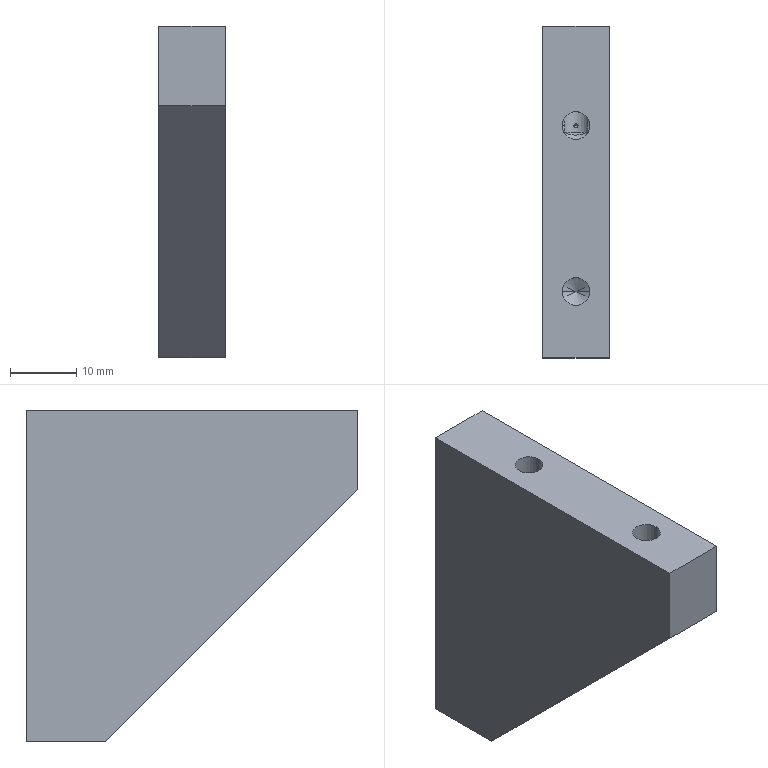Component | SolidWorks | LD101-02--Q1070-Q1-2-2 | 1 solid | 37 faces | box 10 x 50 x 50 mm | volume 16911 mm3 | cone 16 | cylinder 14 | plane 7 | commonest cylinder face diameters 4.2 x14 | material AL6061
STEP:
#1=CARTESIAN_POINT('',(6.957,-10.991,10.561));
#2=VERTEX_POINT('',#1);
#3=CARTESIAN_POINT('',(6.969,-10.983,10.561));
#4=VERTEX_POINT('',#3);
#5=CARTESIAN_POINT('',(7.04,-10.941,10.561));
#6=DIRECTION('',(0.8572,0.515,0.));
#7=VECTOR('',#6,39.37);
#8=LINE('',#5,#7);
#9=EDGE_CURVE('',#2,#4,#8,.T.);
#10=ORIENTED_EDGE('',*,*,#9,.F.);
#11=CARTESIAN_POINT('',(6.945,-10.983,10.561));
#12=VERTEX_POINT('',#11);
#13=CARTESIAN_POINT('',(6.874,-10.941,10.561));
#14=DIRECTION('',(-0.8572,0.515,-0.));
#15=VECTOR('',#14,39.37);
#16=LINE('',#13,#15);
#17=EDGE_CURVE('',#2,#12,#16,.T.);
#18=ORIENTED_EDGE('',*,*,#17,.T.);
#19=CARTESIAN_POINT('',(6.945,-10.983,10.561));
#20=CARTESIAN_POINT('',(6.945,-10.983,10.564));
#21=CARTESIAN_POINT('',(6.947,-10.983,10.567));
#22=CARTESIAN_POINT('',(6.951,-10.984,10.571));
#23=CARTESIAN_POINT('',(6.954,-10.984,10.572));
#24=CARTESIAN_POINT('',(6.96,-10.984,10.572));
#25=CARTESIAN_POINT('',(6.963,-10.984,10.571));
#26=CARTESIAN_POINT('',(6.968,-10.983,10.567));
#27=CARTESIAN_POINT('',(6.969,-10.983,10.564));
#28=CARTESIAN_POINT('',(6.969,-10.983,10.561));
#29=B_SPLINE_CURVE_WITH_KNOTS('',3,(#19,#20,#21,#22,#23,#24,#25,#26,#27,#28),.UNSPECIFIED.,.F.,.F.,(4,2,2,2,4),(0.000232,0.0004572,0.0006825,0.0009077,0.001133),.UNSPECIFIED.);
#30=EDGE_CURVE('',#12,#4,#29,.T.);
#31=ORIENTED_EDGE('',*,*,#30,.T.);
#32=EDGE_LOOP('',(#10,#18,#31));
#33=FACE_OUTER_BOUND('',#32,.T.);
#34=CARTESIAN_POINT('',(6.957,-10.941,10.561));
#35=DIRECTION('',(-0.,1.,-0.));
#36=DIRECTION('',(1.,0.,0.));
#37=AXIS2_PLACEMENT_3D('',#34,#35,#36);
#38=CONICAL_SURFACE('',#37,0.08268,1.03);
#39=ADVANCED_FACE('',(#33),#38,.F.);
#40=CARTESIAN_POINT('',(7.04,-10.941,10.561));
#41=VERTEX_POINT('',#40);
#42=CARTESIAN_POINT('',(7.03,-10.941,10.522));
#43=VERTEX_POINT('',#42);
#44=CARTESIAN_POINT('',(6.957,-10.941,10.561));
#45=DIRECTION('',(-0.,1.,-0.));
#46=DIRECTION('',(1.,0.,0.));
#47=AXIS2_PLACEMENT_3D('',#44,#45,#46);
#48=CIRCLE('',#47,0.08268);
#49=EDGE_CURVE('',#41,#43,#48,.T.);
#50=ORIENTED_EDGE('',*,*,#49,.F.);
#51=CARTESIAN_POINT('',(7.04,-10.901,10.561));
#52=VERTEX_POINT('',#51);
#53=CARTESIAN_POINT('',(7.04,-10.311,10.561));
#54=DIRECTION('',(-0.,1.,-0.));
#55=VECTOR('',#54,39.37);
#56=LINE('',#53,#55);
#57=EDGE_CURVE('',#41,#52,#56,.T.);
#58=ORIENTED_EDGE('',*,*,#57,.T.);
#59=CARTESIAN_POINT('',(7.04,-10.901,10.561));
#60=CARTESIAN_POINT('',(7.04,-10.915,10.547));
#61=CARTESIAN_POINT('',(7.036,-10.929,10.534));
#62=CARTESIAN_POINT('',(7.03,-10.941,10.522));
#63=(BOUNDED_CURVE()B_SPLINE_CURVE(3,(#59,#60,#61,#62),.UNSPECIFIED.,.F.,.F.)B_SPLINE_CURVE_WITH_KNOTS((4,4),(1.571,2.067),.UNSPECIFIED.)CURVE()GEOMETRIC_REPRESENTATION_ITEM()RATIONAL_B_SPLINE_CURVE((1.,0.9796,0.9796,1.))REPRESENTATION_ITEM(''));
#64=EDGE_CURVE('',#52,#43,#63,.T.);
#65=ORIENTED_EDGE('',*,*,#64,.T.);
#66=EDGE_LOOP('',(#50,#58,#65));
#67=FACE_OUTER_BOUND('',#66,.T.);
#68=CARTESIAN_POINT('',(6.957,-10.311,10.561));
#69=DIRECTION('',(-0.,1.,-0.));
#70=DIRECTION('',(1.,0.,0.));
#71=AXIS2_PLACEMENT_3D('',#68,#69,#70);
#72=CYLINDRICAL_SURFACE('',#71,0.08268);
#73=ADVANCED_FACE('',(#67),#72,.F.);
#74=CARTESIAN_POINT('',(7.024,-10.951,10.561));
#75=VERTEX_POINT('',#74);
#76=CARTESIAN_POINT('',(7.03,-10.941,10.522));
#77=CARTESIAN_POINT('',(7.028,-10.943,10.528));
#78=CARTESIAN_POINT('',(7.027,-10.946,10.534));
#79=CARTESIAN_POINT('',(7.025,-10.948,10.544));
#80=CARTESIAN_POINT('',(7.025,-10.949,10.547));
#81=CARTESIAN_POINT('',(7.024,-10.95,10.554));
#82=CARTESIAN_POINT('',(7.024,-10.951,10.558));
#83=CARTESIAN_POINT('',(7.024,-10.951,10.561));
#84=B_SPLINE_CURVE_WITH_KNOTS('',3,(#76,#77,#78,#79,#80,#81,#82,#83),.UNSPECIFIED.,.F.,.F.,(4,2,2,4),(0.0002892,0.00081,0.00107,0.001331),.UNSPECIFIED.);
#85=EDGE_CURVE('',#43,#75,#84,.T.);
#86=ORIENTED_EDGE('',*,*,#85,.T.);
#87=CARTESIAN_POINT('',(7.04,-10.941,10.561));
#88=DIRECTION('',(0.8572,0.515,0.));
#89=VECTOR('',#88,39.37);
#90=LINE('',#87,#89);
#91=EDGE_CURVE('',#75,#41,#90,.T.);
#92=ORIENTED_EDGE('',*,*,#91,.T.);
#93=ORIENTED_EDGE('',*,*,#49,.T.);
#94=EDGE_LOOP('',(#86,#92,#93));
#95=FACE_OUTER_BOUND('',#94,.T.);
#96=CARTESIAN_POINT('',(6.957,-10.941,10.561));
#97=DIRECTION('',(-0.,1.,-0.));
#98=DIRECTION('',(1.,0.,0.));
#99=AXIS2_PLACEMENT_3D('',#96,#97,#98);
#100=CONICAL_SURFACE('',#99,0.08268,1.03);
#101=ADVANCED_FACE('',(#95),#100,.F.);
#102=CARTESIAN_POINT('',(6.874,-10.901,10.561));
#103=VERTEX_POINT('',#102);
#104=CARTESIAN_POINT('',(7.04,-10.901,10.561));
#105=CARTESIAN_POINT('',(7.04,-10.736,10.727));
#106=CARTESIAN_POINT('',(6.874,-10.736,10.727));
#107=CARTESIAN_POINT('',(6.874,-10.901,10.561));
#108=(BOUNDED_CURVE()B_SPLINE_CURVE(3,(#104,#105,#106,#107),.UNSPECIFIED.,.F.,.F.)B_SPLINE_CURVE_WITH_KNOTS((4,4),(4.712,7.854),.UNSPECIFIED.)CURVE()GEOMETRIC_REPRESENTATION_ITEM()RATIONAL_B_SPLINE_CURVE((1.,0.3333,0.3333,1.))REPRESENTATION_ITEM(''));
#109=EDGE_CURVE('',#52,#103,#108,.T.);
#110=ORIENTED_EDGE('',*,*,#109,.F.);
#111=CARTESIAN_POINT('',(7.04,-10.901,11.152));
#112=VERTEX_POINT('',#111);
#113=CARTESIAN_POINT('',(7.04,-10.901,11.152));
#114=DIRECTION('',(-0.,0.,1.));
#115=VECTOR('',#114,39.37);
#116=LINE('',#113,#115);
#117=EDGE_CURVE('',#52,#112,#116,.T.);
#118=ORIENTED_EDGE('',*,*,#117,.T.);
#119=CARTESIAN_POINT('',(6.874,-10.901,11.152));
#120=VERTEX_POINT('',#119);
#121=CARTESIAN_POINT('',(6.957,-10.901,11.152));
#122=DIRECTION('',(-0.,0.,1.));
#123=DIRECTION('',(-1.,0.,0.));
#124=AXIS2_PLACEMENT_3D('',#121,#122,#123);
#125=CIRCLE('',#124,0.08268);
#126=EDGE_CURVE('',#112,#120,#125,.T.);
#127=ORIENTED_EDGE('',*,*,#126,.T.);
#128=CARTESIAN_POINT('',(6.874,-10.901,11.152));
#129=DIRECTION('',(-0.,0.,1.));
#130=VECTOR('',#129,39.37);
#131=LINE('',#128,#130);
#132=EDGE_CURVE('',#103,#120,#131,.T.);
#133=ORIENTED_EDGE('',*,*,#132,.F.);
#134=EDGE_LOOP('',(#110,#118,#127,#133));
#135=FACE_OUTER_BOUND('',#134,.T.);
#136=CARTESIAN_POINT('',(6.957,-10.901,11.152));
#137=DIRECTION('',(-0.,0.,1.));
#138=DIRECTION('',(-1.,0.,0.));
#139=AXIS2_PLACEMENT_3D('',#136,#137,#138);
#140=CYLINDRICAL_SURFACE('',#139,0.08268);
#141=ADVANCED_FACE('',(#135),#140,.F.);
#142=CARTESIAN_POINT('',(6.874,-10.901,10.522));
#143=VERTEX_POINT('',#142);
#144=CARTESIAN_POINT('',(6.884,-10.941,10.522));
#145=VERTEX_POINT('',#144);
#146=CARTESIAN_POINT('',(6.957,-10.901,10.522));
#147=DIRECTION('',(-0.,0.,1.));
#148=DIRECTION('',(-1.,0.,0.));
#149=AXIS2_PLACEMENT_3D('',#146,#147,#148);
#150=CIRCLE('',#149,0.08268);
#151=EDGE_CURVE('',#143,#145,#150,.T.);
#152=ORIENTED_EDGE('',*,*,#151,.F.);
#153=CARTESIAN_POINT('',(6.874,-10.901,11.152));
#154=DIRECTION('',(-0.,0.,1.));
#155=VECTOR('',#154,39.37);
#156=LINE('',#153,#155);
#157=EDGE_CURVE('',#143,#103,#156,.T.);
#158=ORIENTED_EDGE('',*,*,#157,.T.);
#159=CARTESIAN_POINT('',(6.884,-10.941,10.522));
#160=CARTESIAN_POINT('',(6.878,-10.929,10.534));
#161=CARTESIAN_POINT('',(6.874,-10.915,10.547));
#162=CARTESIAN_POINT('',(6.874,-10.901,10.561));
#163=(BOUNDED_CURVE()B_SPLINE_CURVE(3,(#159,#160,#161,#162),.UNSPECIFIED.,.F.,.F.)B_SPLINE_CURVE_WITH_KNOTS((4,4),(4.216,4.712),.UNSPECIFIED.)CURVE()GEOMETRIC_REPRESENTATION_ITEM()RATIONAL_B_SPLINE_CURVE((1.,0.9796,0.9796,1.))REPRESENTATION_ITEM(''));
#164=EDGE_CURVE('',#145,#103,#163,.T.);
#165=ORIENTED_EDGE('',*,*,#164,.F.);
#166=EDGE_LOOP('',(#152,#158,#165));
#167=FACE_OUTER_BOUND('',#166,.T.);
#168=CARTESIAN_POINT('',(6.957,-10.901,11.152));
#169=DIRECTION('',(-0.,0.,1.));
#170=DIRECTION('',(-1.,0.,0.));
#171=AXIS2_PLACEMENT_3D('',#168,#169,#170);
#172=CYLINDRICAL_SURFACE('',#171,0.08268);
#173=ADVANCED_FACE('',(#167),#172,.F.);
#174=CARTESIAN_POINT('',(6.891,-10.901,10.512));
#175=VERTEX_POINT('',#174);
#176=CARTESIAN_POINT('',(6.891,-10.901,10.512));
#177=CARTESIAN_POINT('',(6.891,-10.908,10.512));
#178=CARTESIAN_POINT('',(6.89,-10.915,10.513));
#179=CARTESIAN_POINT('',(6.887,-10.928,10.517));
#180=CARTESIAN_POINT('',(6.886,-10.935,10.519));
#181=CARTESIAN_POINT('',(6.884,-10.941,10.522));
#182=B_SPLINE_CURVE_WITH_KNOTS('',3,(#176,#177,#178,#179,#180,#181),.UNSPECIFIED.,.F.,.F.,(4,2,4),(0.001331,0.001845,0.00236),.UNSPECIFIED.);
#183=EDGE_CURVE('',#175,#145,#182,.T.);
#184=ORIENTED_EDGE('',*,*,#183,.F.);
#185=CARTESIAN_POINT('',(6.874,-10.901,10.522));
#186=DIRECTION('',(-0.8572,0.,0.515));
#187=VECTOR('',#186,39.37);
#188=LINE('',#185,#187);
#189=EDGE_CURVE('',#175,#143,#188,.T.);
#190=ORIENTED_EDGE('',*,*,#189,.T.);
#191=ORIENTED_EDGE('',*,*,#151,.T.);
#192=EDGE_LOOP('',(#184,#190,#191));
#193=FACE_OUTER_BOUND('',#192,.T.);
#194=CARTESIAN_POINT('',(6.957,-10.901,10.522));
#195=DIRECTION('',(-0.,0.,1.));
#196=DIRECTION('',(-1.,0.,0.));
#197=AXIS2_PLACEMENT_3D('',#194,#195,#196);
#198=CONICAL_SURFACE('',#197,0.08268,1.03);
#199=ADVANCED_FACE('',(#193),#198,.F.);
#200=CARTESIAN_POINT('',(6.957,-10.901,10.472));
#201=VERTEX_POINT('',#200);
#202=CARTESIAN_POINT('',(6.945,-10.901,10.479));
#203=VERTEX_POINT('',#202);
#204=CARTESIAN_POINT('',(6.874,-10.901,10.522));
#205=DIRECTION('',(-0.8572,0.,0.515));
#206=VECTOR('',#205,39.37);
#207=LINE('',#204,#206);
#208=EDGE_CURVE('',#201,#203,#207,.T.);
#209=ORIENTED_EDGE('',*,*,#208,.F.);
#210=CARTESIAN_POINT('',(6.969,-10.901,10.479));
#211=VERTEX_POINT('',#210);
#212=CARTESIAN_POINT('',(7.04,-10.901,10.522));
#213=DIRECTION('',(0.8572,0.,0.515));
#214=VECTOR('',#213,39.37);
#215=LINE('',#212,#214);
#216=EDGE_CURVE('',#201,#211,#215,.T.);
#217=ORIENTED_EDGE('',*,*,#216,.T.);
#218=CARTESIAN_POINT('',(6.945,-10.901,10.479));
#219=CARTESIAN_POINT('',(6.945,-10.898,10.479));
#220=CARTESIAN_POINT('',(6.947,-10.896,10.479));
#221=CARTESIAN_POINT('',(6.951,-10.892,10.479));
#222=CARTESIAN_POINT('',(6.954,-10.891,10.479));
#223=CARTESIAN_POINT('',(6.96,-10.891,10.479));
#224=CARTESIAN_POINT('',(6.963,-10.892,10.479));
#225=CARTESIAN_POINT('',(6.968,-10.896,10.479));
#226=CARTESIAN_POINT('',(6.969,-10.898,10.479));
#227=CARTESIAN_POINT('',(6.969,-10.901,10.479));
#228=B_SPLINE_CURVE_WITH_KNOTS('',3,(#218,#219,#220,#221,#222,#223,#224,#225,#226,#227),.UNSPECIFIED.,.F.,.F.,(4,2,2,2,4),(0.000232,0.0004572,0.0006825,0.0009077,0.001133),.UNSPECIFIED.);
#229=EDGE_CURVE('',#203,#211,#228,.T.);
#230=ORIENTED_EDGE('',*,*,#229,.F.);
#231=EDGE_LOOP('',(#209,#217,#230));
#232=FACE_OUTER_BOUND('',#231,.T.);
#233=CARTESIAN_POINT('',(6.957,-10.901,10.522));
#234=DIRECTION('',(-0.,0.,1.));
#235=DIRECTION('',(-1.,0.,0.));
#236=AXIS2_PLACEMENT_3D('',#233,#234,#235);
#237=CONICAL_SURFACE('',#236,0.08268,1.03);
#238=ADVANCED_FACE('',(#232),#237,.F.);
#239=CARTESIAN_POINT('',(7.04,-11.886,10.522));
#240=VERTEX_POINT('',#239);
#241=CARTESIAN_POINT('',(6.874,-11.886,10.522));
#242=VERTEX_POINT('',#241);
#243=CARTESIAN_POINT('',(6.957,-11.886,10.522));
#244=DIRECTION('',(-0.,0.,1.));
#245=DIRECTION('',(-1.,0.,0.));
#246=AXIS2_PLACEMENT_3D('',#243,#244,#245);
#247=CIRCLE('',#246,0.08268);
#248=EDGE_CURVE('',#240,#242,#247,.T.);
#249=ORIENTED_EDGE('',*,*,#248,.F.);
#250=CARTESIAN_POINT('',(7.04,-11.886,11.152));
#251=VERTEX_POINT('',#250);
#252=CARTESIAN_POINT('',(7.04,-11.886,11.152));
#253=DIRECTION('',(-0.,0.,1.));
#254=VECTOR('',#253,39.37);
#255=LINE('',#252,#254);
#256=EDGE_CURVE('',#240,#251,#255,.T.);
#257=ORIENTED_EDGE('',*,*,#256,.T.);
#258=CARTESIAN_POINT('',(6.874,-11.886,11.152));
#259=VERTEX_POINT('',#258);
#260=CARTESIAN_POINT('',(6.957,-11.886,11.152));
#261=DIRECTION('',(-0.,0.,1.));
#262=DIRECTION('',(-1.,0.,0.));
#263=AXIS2_PLACEMENT_3D('',#260,#261,#262);
#264=CIRCLE('',#263,0.08268);
#265=EDGE_CURVE('',#251,#259,#264,.T.);
#266=ORIENTED_EDGE('',*,*,#265,.T.);
#267=CARTESIAN_POINT('',(6.874,-11.886,11.152));
#268=DIRECTION('',(-0.,0.,1.));
#269=VECTOR('',#268,39.37);
#270=LINE('',#267,#269);
#271=EDGE_CURVE('',#242,#259,#270,.T.);
#272=ORIENTED_EDGE('',*,*,#271,.F.);
#273=EDGE_LOOP('',(#249,#257,#266,#272));
#274=FACE_OUTER_BOUND('',#273,.T.);
#275=CARTESIAN_POINT('',(6.957,-11.886,11.152));
#276=DIRECTION('',(-0.,0.,1.));
#277=DIRECTION('',(-1.,0.,0.));
#278=AXIS2_PLACEMENT_3D('',#275,#276,#277);
#279=CYLINDRICAL_SURFACE('',#278,0.08268);
#280=ADVANCED_FACE('',(#274),#279,.F.);
#281=CARTESIAN_POINT('',(6.957,-11.886,10.472));
#282=VERTEX_POINT('',#281);
#283=CARTESIAN_POINT('',(6.874,-11.886,10.522));
#284=DIRECTION('',(-0.8572,0.,0.515));
#285=VECTOR('',#284,39.37);
#286=LINE('',#283,#285);
#287=EDGE_CURVE('',#282,#242,#286,.T.);
#288=ORIENTED_EDGE('',*,*,#287,.F.);
#289=CARTESIAN_POINT('',(7.04,-11.886,10.522));
#290=DIRECTION('',(0.8572,0.,0.515));
#291=VECTOR('',#290,39.37);
#292=LINE('',#289,#291);
#293=EDGE_CURVE('',#282,#240,#292,.T.);
#294=ORIENTED_EDGE('',*,*,#293,.T.);
#295=ORIENTED_EDGE('',*,*,#248,.T.);
#296=EDGE_LOOP('',(#288,#294,#295));
#297=FACE_OUTER_BOUND('',#296,.T.);
#298=CARTESIAN_POINT('',(6.957,-11.886,10.522));
#299=DIRECTION('',(-0.,0.,1.));
#300=DIRECTION('',(-1.,0.,0.));
#301=AXIS2_PLACEMENT_3D('',#298,#299,#300);
#302=CONICAL_SURFACE('',#301,0.08268,1.03);
#303=ADVANCED_FACE('',(#297),#302,.F.);
#304=CARTESIAN_POINT('',(6.874,-10.941,9.577));
#305=VERTEX_POINT('',#304);
#306=CARTESIAN_POINT('',(7.04,-10.941,9.577));
#307=VERTEX_POINT('',#306);
#308=CARTESIAN_POINT('',(6.957,-10.941,9.577));
#309=DIRECTION('',(-0.,1.,-0.));
#310=DIRECTION('',(1.,0.,0.));
#311=AXIS2_PLACEMENT_3D('',#308,#309,#310);
#312=CIRCLE('',#311,0.08268);
#313=EDGE_CURVE('',#305,#307,#312,.T.);
#314=ORIENTED_EDGE('',*,*,#313,.F.);
#315=CARTESIAN_POINT('',(6.874,-10.311,9.577));
#316=VERTEX_POINT('',#315);
#317=CARTESIAN_POINT('',(6.874,-10.311,9.577));
#318=DIRECTION('',(-0.,1.,-0.));
#319=VECTOR('',#318,39.37);
#320=LINE('',#317,#319);
#321=EDGE_CURVE('',#305,#316,#320,.T.);
#322=ORIENTED_EDGE('',*,*,#321,.T.);
#323=CARTESIAN_POINT('',(7.04,-10.311,9.577));
#324=VERTEX_POINT('',#323);
#325=CARTESIAN_POINT('',(6.957,-10.311,9.577));
#326=DIRECTION('',(-0.,1.,-0.));
#327=DIRECTION('',(1.,0.,0.));
#328=AXIS2_PLACEMENT_3D('',#325,#326,#327);
#329=CIRCLE('',#328,0.08268);
#330=EDGE_CURVE('',#316,#324,#329,.T.);
#331=ORIENTED_EDGE('',*,*,#330,.T.);
#332=CARTESIAN_POINT('',(7.04,-10.311,9.577));
#333=DIRECTION('',(-0.,1.,-0.));
#334=VECTOR('',#333,39.37);
#335=LINE('',#332,#334);
#336=EDGE_CURVE('',#307,#324,#335,.T.);
#337=ORIENTED_EDGE('',*,*,#336,.F.);
#338=EDGE_LOOP('',(#314,#322,#331,#337));
#339=FACE_OUTER_BOUND('',#338,.T.);
#340=CARTESIAN_POINT('',(6.957,-10.311,9.577));
#341=DIRECTION('',(-0.,1.,-0.));
#342=DIRECTION('',(1.,0.,0.));
#343=AXIS2_PLACEMENT_3D('',#340,#341,#342);
#344=CYLINDRICAL_SURFACE('',#343,0.08268);
#345=ADVANCED_FACE('',(#339),#344,.F.);
#346=CARTESIAN_POINT('',(6.957,-10.991,9.577));
#347=VERTEX_POINT('',#346);
#348=CARTESIAN_POINT('',(7.04,-10.941,9.577));
#349=DIRECTION('',(0.8572,0.515,0.));
#350=VECTOR('',#349,39.37);
#351=LINE('',#348,#350);
#352=EDGE_CURVE('',#347,#307,#351,.T.);
#353=ORIENTED_EDGE('',*,*,#352,.F.);
#354=CARTESIAN_POINT('',(6.874,-10.941,9.577));
#355=DIRECTION('',(-0.8572,0.515,-0.));
#356=VECTOR('',#355,39.37);
#357=LINE('',#354,#356);
#358=EDGE_CURVE('',#347,#305,#357,.T.);
#359=ORIENTED_EDGE('',*,*,#358,.T.);
#360=ORIENTED_EDGE('',*,*,#313,.T.);
#361=EDGE_LOOP('',(#353,#359,#360));
#362=FACE_OUTER_BOUND('',#361,.T.);
#363=CARTESIAN_POINT('',(6.957,-10.941,9.577));
#364=DIRECTION('',(-0.,1.,-0.));
#365=DIRECTION('',(1.,0.,0.));
#366=AXIS2_PLACEMENT_3D('',#363,#364,#365);
#367=CONICAL_SURFACE('',#366,0.08268,1.03);
#368=ADVANCED_FACE('',(#362),#367,.F.);
#369=ORIENTED_EDGE('',*,*,#109,.T.);
#370=CARTESIAN_POINT('',(6.874,-10.311,10.561));
#371=VERTEX_POINT('',#370);
#372=CARTESIAN_POINT('',(6.874,-10.311,10.561));
#373=DIRECTION('',(-0.,1.,-0.));
#374=VECTOR('',#373,39.37);
#375=LINE('',#372,#374);
#376=EDGE_CURVE('',#103,#371,#375,.T.);
#377=ORIENTED_EDGE('',*,*,#376,.T.);
#378=CARTESIAN_POINT('',(7.04,-10.311,10.561));
#379=VERTEX_POINT('',#378);
#380=CARTESIAN_POINT('',(6.957,-10.311,10.561));
#381=DIRECTION('',(-0.,1.,-0.));
#382=DIRECTION('',(1.,0.,0.));
#383=AXIS2_PLACEMENT_3D('',#380,#381,#382);
#384=CIRCLE('',#383,0.08268);
#385=EDGE_CURVE('',#371,#379,#384,.T.);
#386=ORIENTED_EDGE('',*,*,#385,.T.);
#387=CARTESIAN_POINT('',(7.04,-10.311,10.561));
#388=DIRECTION('',(-0.,1.,-0.));
#389=VECTOR('',#388,39.37);
#390=LINE('',#387,#389);
#391=EDGE_CURVE('',#52,#379,#390,.T.);
#392=ORIENTED_EDGE('',*,*,#391,.F.);
#393=EDGE_LOOP('',(#369,#377,#386,#392));
#394=FACE_OUTER_BOUND('',#393,.T.);
#395=CARTESIAN_POINT('',(6.957,-10.311,10.561));
#396=DIRECTION('',(-0.,1.,-0.));
#397=DIRECTION('',(1.,0.,0.));
#398=AXIS2_PLACEMENT_3D('',#395,#396,#397);
#399=CYLINDRICAL_SURFACE('',#398,0.08268);
#400=ADVANCED_FACE('',(#394),#399,.F.);
#401=CARTESIAN_POINT('',(6.957,-10.941,10.561));
#402=DIRECTION('',(-0.,1.,-0.));
#403=DIRECTION('',(1.,0.,0.));
#404=AXIS2_PLACEMENT_3D('',#401,#402,#403);
#405=CIRCLE('',#404,0.08268);
#406=EDGE_CURVE('',#43,#145,#405,.T.);
#407=ORIENTED_EDGE('',*,*,#406,.T.);
#408=CARTESIAN_POINT('',(6.884,-10.941,10.522));
#409=CARTESIAN_POINT('',(6.896,-10.945,10.517));
#410=CARTESIAN_POINT('',(6.907,-10.949,10.513));
#411=CARTESIAN_POINT('',(6.925,-10.954,10.509));
#412=CARTESIAN_POINT('',(6.931,-10.955,10.508));
#413=CARTESIAN_POINT('',(6.944,-10.957,10.506));
#414=CARTESIAN_POINT('',(6.951,-10.957,10.506));
#415=CARTESIAN_POINT('',(6.963,-10.957,10.506));
#416=CARTESIAN_POINT('',(6.97,-10.957,10.506));
#417=CARTESIAN_POINT('',(6.983,-10.955,10.508));
#418=CARTESIAN_POINT('',(6.989,-10.954,10.509));
#419=CARTESIAN_POINT('',(7.007,-10.949,10.513));
#420=CARTESIAN_POINT('',(7.019,-10.945,10.517));
#421=CARTESIAN_POINT('',(7.03,-10.941,10.522));
#422=B_SPLINE_CURVE_WITH_KNOTS('',3,(#408,#409,#410,#411,#412,#413,#414,#415,#416,#417,#418,#419,#420,#421),.UNSPECIFIED.,.F.,.F.,(4,2,2,2,2,2,4),(0.00000056,0.00097,0.001455,0.001939,0.002424,0.002909,0.003878),.UNSPECIFIED.);
#423=EDGE_CURVE('',#145,#43,#422,.T.);
#424=ORIENTED_EDGE('',*,*,#423,.T.);
#425=EDGE_LOOP('',(#407,#424));
#426=FACE_OUTER_BOUND('',#425,.T.);
#427=CARTESIAN_POINT('',(6.957,-10.941,10.561));
#428=DIRECTION('',(-0.,1.,-0.));
#429=DIRECTION('',(1.,0.,0.));
#430=AXIS2_PLACEMENT_3D('',#427,#428,#429);
#431=CONICAL_SURFACE('',#430,0.08268,1.03);
#432=ADVANCED_FACE('',(#426),#431,.F.);
#433=ORIENTED_EDGE('',*,*,#376,.F.);
#434=CARTESIAN_POINT('',(6.884,-10.862,10.522));
#435=VERTEX_POINT('',#434);
#436=CARTESIAN_POINT('',(6.874,-10.901,10.561));
#437=CARTESIAN_POINT('',(6.874,-10.888,10.547));
#438=CARTESIAN_POINT('',(6.878,-10.874,10.534));
#439=CARTESIAN_POINT('',(6.884,-10.862,10.522));
#440=(BOUNDED_CURVE()B_SPLINE_CURVE(3,(#436,#437,#438,#439),.UNSPECIFIED.,.F.,.T.)B_SPLINE_CURVE_WITH_KNOTS((4,4),(4.712,5.209),.UNSPECIFIED.)CURVE()GEOMETRIC_REPRESENTATION_ITEM()RATIONAL_B_SPLINE_CURVE((1.,0.9796,0.9796,1.))REPRESENTATION_ITEM(''));
#441=EDGE_CURVE('',#103,#435,#440,.T.);
#442=ORIENTED_EDGE('',*,*,#441,.T.);
#443=CARTESIAN_POINT('',(6.884,-10.862,10.522));
#444=CARTESIAN_POINT('',(6.886,-10.868,10.519));
#445=CARTESIAN_POINT('',(6.887,-10.875,10.517));
#446=CARTESIAN_POINT('',(6.889,-10.884,10.514));
#447=CARTESIAN_POINT('',(6.89,-10.888,10.514));
#448=CARTESIAN_POINT('',(6.89,-10.894,10.513));
#449=CARTESIAN_POINT('',(6.891,-10.898,10.512));
#450=CARTESIAN_POINT('',(6.891,-10.901,10.512));
#451=B_SPLINE_CURVE_WITH_KNOTS('',3,(#443,#444,#445,#446,#447,#448,#449,#450),.UNSPECIFIED.,.F.,.F.,(4,2,2,4),(0.0002892,0.00081,0.00107,0.001331),.UNSPECIFIED.);
#452=EDGE_CURVE('',#435,#175,#451,.T.);
#453=ORIENTED_EDGE('',*,*,#452,.T.);
#454=ORIENTED_EDGE('',*,*,#183,.T.);
#455=ORIENTED_EDGE('',*,*,#406,.F.);
#456=CARTESIAN_POINT('',(7.03,-10.862,10.522));
#457=VERTEX_POINT('',#456);
#458=CARTESIAN_POINT('',(7.03,-10.941,10.522));
#459=CARTESIAN_POINT('',(7.028,-10.935,10.519));
#460=CARTESIAN_POINT('',(7.027,-10.928,10.517));
#461=CARTESIAN_POINT('',(7.025,-10.919,10.514));
#462=CARTESIAN_POINT('',(7.025,-10.915,10.514));
#463=CARTESIAN_POINT('',(7.024,-10.909,10.513));
#464=CARTESIAN_POINT('',(7.024,-10.905,10.512));
#465=CARTESIAN_POINT('',(7.024,-10.895,10.512));
#466=CARTESIAN_POINT('',(7.025,-10.888,10.513));
#467=CARTESIAN_POINT('',(7.027,-10.875,10.517));
#468=CARTESIAN_POINT('',(7.028,-10.868,10.519));
#469=CARTESIAN_POINT('',(7.03,-10.862,10.522));
#470=B_SPLINE_CURVE_WITH_KNOTS('',3,(#458,#459,#460,#461,#462,#463,#464,#465,#466,#467,#468,#469),.UNSPECIFIED.,.F.,.F.,(4,2,2,2,2,4),(0.0002892,0.0008068,0.001066,0.001324,0.001842,0.00236),.UNSPECIFIED.);
#471=EDGE_CURVE('',#43,#457,#470,.T.);
#472=ORIENTED_EDGE('',*,*,#471,.T.);
#473=CARTESIAN_POINT('',(7.03,-10.862,10.522));
#474=CARTESIAN_POINT('',(7.036,-10.874,10.534));
#475=CARTESIAN_POINT('',(7.04,-10.888,10.547));
#476=CARTESIAN_POINT('',(7.04,-10.901,10.561));
#477=(BOUNDED_CURVE()B_SPLINE_CURVE(3,(#473,#474,#475,#476),.UNSPECIFIED.,.F.,.F.)B_SPLINE_CURVE_WITH_KNOTS((4,4),(1.074,1.571),.UNSPECIFIED.)CURVE()GEOMETRIC_REPRESENTATION_ITEM()RATIONAL_B_SPLINE_CURVE((1.,0.9796,0.9796,1.))REPRESENTATION_ITEM(''));
#478=EDGE_CURVE('',#457,#52,#477,.T.);
#479=ORIENTED_EDGE('',*,*,#478,.T.);
#480=ORIENTED_EDGE('',*,*,#391,.T.);
#481=CARTESIAN_POINT('',(6.957,-10.311,10.561));
#482=DIRECTION('',(-0.,1.,-0.));
#483=DIRECTION('',(1.,0.,0.));
#484=AXIS2_PLACEMENT_3D('',#481,#482,#483);
#485=CIRCLE('',#484,0.08268);
#486=EDGE_CURVE('',#379,#371,#485,.T.);
#487=ORIENTED_EDGE('',*,*,#486,.T.);
#488=EDGE_LOOP('',(#433,#442,#453,#454,#455,#472,#479,#480,#487));
#489=FACE_OUTER_BOUND('',#488,.T.);
#490=ORIENTED_EDGE('',*,*,#229,.T.);
#491=CARTESIAN_POINT('',(6.969,-10.901,10.479));
#492=CARTESIAN_POINT('',(6.969,-10.904,10.479));
#493=CARTESIAN_POINT('',(6.968,-10.907,10.479));
#494=CARTESIAN_POINT('',(6.963,-10.911,10.479));
#495=CARTESIAN_POINT('',(6.96,-10.912,10.479));
#496=CARTESIAN_POINT('',(6.954,-10.912,10.479));
#497=CARTESIAN_POINT('',(6.951,-10.911,10.479));
#498=CARTESIAN_POINT('',(6.947,-10.907,10.479));
#499=CARTESIAN_POINT('',(6.945,-10.904,10.479));
#500=CARTESIAN_POINT('',(6.945,-10.901,10.479));
#501=B_SPLINE_CURVE_WITH_KNOTS('',3,(#491,#492,#493,#494,#495,#496,#497,#498,#499,#500),.UNSPECIFIED.,.F.,.F.,(4,2,2,2,4),(0.001133,0.001358,0.001583,0.001807,0.002032),.UNSPECIFIED.);
#502=EDGE_CURVE('',#211,#203,#501,.T.);
#503=ORIENTED_EDGE('',*,*,#502,.T.);
#504=EDGE_LOOP('',(#490,#503));
#505=FACE_BOUND('',#504,.T.);
#506=CARTESIAN_POINT('',(6.957,-10.311,10.561));
#507=DIRECTION('',(-0.,1.,-0.));
#508=DIRECTION('',(1.,0.,0.));
#509=AXIS2_PLACEMENT_3D('',#506,#507,#508);
#510=CYLINDRICAL_SURFACE('',#509,0.08268);
#511=ADVANCED_FACE('',(#489,#505),#510,.F.);
#512=ORIENTED_EDGE('',*,*,#486,.F.);
#513=ORIENTED_EDGE('',*,*,#385,.F.);
#514=EDGE_LOOP('',(#512,#513));
#515=FACE_BOUND('',#514,.T.);
#516=CARTESIAN_POINT('',(6.957,-10.311,9.577));
#517=DIRECTION('',(-0.,1.,-0.));
#518=DIRECTION('',(1.,0.,0.));
#519=AXIS2_PLACEMENT_3D('',#516,#517,#518);
#520=CIRCLE('',#519,0.08268);
#521=EDGE_CURVE('',#324,#316,#520,.T.);
#522=ORIENTED_EDGE('',*,*,#521,.F.);
#523=ORIENTED_EDGE('',*,*,#330,.F.);
#524=EDGE_LOOP('',(#522,#523));
#525=FACE_BOUND('',#524,.T.);
#526=CARTESIAN_POINT('',(6.76,-10.311,9.183));
#527=VERTEX_POINT('',#526);
#528=CARTESIAN_POINT('',(6.76,-10.311,11.152));
#529=VERTEX_POINT('',#528);
#530=CARTESIAN_POINT('',(6.76,-10.311,9.183));
#531=DIRECTION('',(-0.,0.,1.));
#532=VECTOR('',#531,39.37);
#533=LINE('',#530,#532);
#534=EDGE_CURVE('',#527,#529,#533,.T.);
#535=ORIENTED_EDGE('',*,*,#534,.T.);
#536=CARTESIAN_POINT('',(7.154,-10.311,11.152));
#537=VERTEX_POINT('',#536);
#538=CARTESIAN_POINT('',(7.154,-10.311,11.152));
#539=DIRECTION('',(-1.,-0.,-0.));
#540=VECTOR('',#539,39.37);
#541=LINE('',#538,#540);
#542=EDGE_CURVE('',#537,#529,#541,.T.);
#543=ORIENTED_EDGE('',*,*,#542,.F.);
#544=CARTESIAN_POINT('',(7.154,-10.311,9.183));
#545=VERTEX_POINT('',#544);
#546=CARTESIAN_POINT('',(7.154,-10.311,9.183));
#547=DIRECTION('',(-0.,0.,1.));
#548=VECTOR('',#547,39.37);
#549=LINE('',#546,#548);
#550=EDGE_CURVE('',#545,#537,#549,.T.);
#551=ORIENTED_EDGE('',*,*,#550,.F.);
#552=CARTESIAN_POINT('',(7.154,-10.311,9.183));
#553=DIRECTION('',(-1.,-0.,-0.));
#554=VECTOR('',#553,39.37);
#555=LINE('',#552,#554);
#556=EDGE_CURVE('',#545,#527,#555,.T.);
#557=ORIENTED_EDGE('',*,*,#556,.T.);
#558=EDGE_LOOP('',(#535,#543,#551,#557));
#559=FACE_OUTER_BOUND('',#558,.T.);
#560=CARTESIAN_POINT('',(7.154,-10.311,9.183));
#561=DIRECTION('',(0.,-1.,0.));
#562=DIRECTION('',(0.,-0.,-1.));
#563=AXIS2_PLACEMENT_3D('',#560,#561,#562);
#564=PLANE('',#563);
#565=ADVANCED_FACE('',(#515,#525,#559),#564,.F.);
#566=CARTESIAN_POINT('',(6.957,-10.901,11.152));
#567=DIRECTION('',(-0.,0.,1.));
#568=DIRECTION('',(-1.,0.,0.));
#569=AXIS2_PLACEMENT_3D('',#566,#567,#568);
#570=CIRCLE('',#569,0.08268);
#571=EDGE_CURVE('',#120,#112,#570,.T.);
#572=ORIENTED_EDGE('',*,*,#571,.F.);
#573=ORIENTED_EDGE('',*,*,#126,.F.);
#574=EDGE_LOOP('',(#572,#573));
#575=FACE_BOUND('',#574,.T.);
#576=CARTESIAN_POINT('',(6.957,-11.886,11.152));
#577=DIRECTION('',(-0.,0.,1.));
#578=DIRECTION('',(-1.,0.,0.));
#579=AXIS2_PLACEMENT_3D('',#576,#577,#578);
#580=CIRCLE('',#579,0.08268);
#581=EDGE_CURVE('',#259,#251,#580,.T.);
#582=ORIENTED_EDGE('',*,*,#581,.F.);
#583=ORIENTED_EDGE('',*,*,#265,.F.);
#584=EDGE_LOOP('',(#582,#583));
#585=FACE_BOUND('',#584,.T.);
#586=CARTESIAN_POINT('',(6.76,-12.279,11.152));
#587=VERTEX_POINT('',#586);
#588=CARTESIAN_POINT('',(6.76,-10.311,11.152));
#589=DIRECTION('',(0.,-1.,0.));
#590=VECTOR('',#589,39.37);
#591=LINE('',#588,#590);
#592=EDGE_CURVE('',#529,#587,#591,.T.);
#593=ORIENTED_EDGE('',*,*,#592,.T.);
#594=CARTESIAN_POINT('',(7.154,-12.279,11.152));
#595=VERTEX_POINT('',#594);
#596=CARTESIAN_POINT('',(7.154,-12.279,11.152));
#597=DIRECTION('',(-1.,-0.,-0.));
#598=VECTOR('',#597,39.37);
#599=LINE('',#596,#598);
#600=EDGE_CURVE('',#595,#587,#599,.T.);
#601=ORIENTED_EDGE('',*,*,#600,.F.);
#602=CARTESIAN_POINT('',(7.154,-10.311,11.152));
#603=DIRECTION('',(0.,-1.,0.));
#604=VECTOR('',#603,39.37);
#605=LINE('',#602,#604);
#606=EDGE_CURVE('',#537,#595,#605,.T.);
#607=ORIENTED_EDGE('',*,*,#606,.F.);
#608=ORIENTED_EDGE('',*,*,#542,.T.);
#609=EDGE_LOOP('',(#593,#601,#607,#608));
#610=FACE_OUTER_BOUND('',#609,.T.);
#611=CARTESIAN_POINT('',(7.154,-10.311,11.152));
#612=DIRECTION('',(0.,-0.,-1.));
#613=DIRECTION('',(1.,0.,0.));
#614=AXIS2_PLACEMENT_3D('',#611,#612,#613);
#615=PLANE('',#614);
#616=ADVANCED_FACE('',(#575,#585,#610),#615,.F.);
#617=CARTESIAN_POINT('',(6.76,-12.279,10.679));
#618=VERTEX_POINT('',#617);
#619=CARTESIAN_POINT('',(6.76,-12.279,11.152));
#620=DIRECTION('',(0.,-0.,-1.));
#621=VECTOR('',#620,39.37);
#622=LINE('',#619,#621);
#623=EDGE_CURVE('',#587,#618,#622,.T.);
#624=ORIENTED_EDGE('',*,*,#623,.T.);
#625=CARTESIAN_POINT('',(7.154,-12.279,10.679));
#626=VERTEX_POINT('',#625);
#627=CARTESIAN_POINT('',(7.154,-12.279,10.679));
#628=DIRECTION('',(-1.,-0.,-0.));
#629=VECTOR('',#628,39.37);
#630=LINE('',#627,#629);
#631=EDGE_CURVE('',#626,#618,#630,.T.);
#632=ORIENTED_EDGE('',*,*,#631,.F.);
#633=CARTESIAN_POINT('',(7.154,-12.279,11.152));
#634=DIRECTION('',(0.,-0.,-1.));
#635=VECTOR('',#634,39.37);
#636=LINE('',#633,#635);
#637=EDGE_CURVE('',#595,#626,#636,.T.);
#638=ORIENTED_EDGE('',*,*,#637,.F.);
#639=ORIENTED_EDGE('',*,*,#600,.T.);
#640=EDGE_LOOP('',(#624,#632,#638,#639));
#641=FACE_OUTER_BOUND('',#640,.T.);
#642=CARTESIAN_POINT('',(7.154,-12.279,11.152));
#643=DIRECTION('',(-0.,1.,-0.));
#644=DIRECTION('',(1.,0.,0.));
#645=AXIS2_PLACEMENT_3D('',#642,#643,#644);
#646=PLANE('',#645);
#647=ADVANCED_FACE('',(#641),#646,.F.);
#648=CARTESIAN_POINT('',(6.76,-10.783,9.183));
#649=VERTEX_POINT('',#648);
#650=CARTESIAN_POINT('',(6.76,-12.279,10.679));
#651=DIRECTION('',(0.,0.7071,-0.7071));
#652=VECTOR('',#651,39.37);
#653=LINE('',#650,#652);
#654=EDGE_CURVE('',#618,#649,#653,.T.);
#655=ORIENTED_EDGE('',*,*,#654,.T.);
#656=CARTESIAN_POINT('',(7.154,-10.783,9.183));
#657=VERTEX_POINT('',#656);
#658=CARTESIAN_POINT('',(7.154,-10.783,9.183));
#659=DIRECTION('',(-1.,-0.,-0.));
#660=VECTOR('',#659,39.37);
#661=LINE('',#658,#660);
#662=EDGE_CURVE('',#657,#649,#661,.T.);
#663=ORIENTED_EDGE('',*,*,#662,.F.);
#664=CARTESIAN_POINT('',(7.154,-12.279,10.679));
#665=DIRECTION('',(0.,0.7071,-0.7071));
#666=VECTOR('',#665,39.37);
#667=LINE('',#664,#666);
#668=EDGE_CURVE('',#626,#657,#667,.T.);
#669=ORIENTED_EDGE('',*,*,#668,.F.);
#670=ORIENTED_EDGE('',*,*,#631,.T.);
#671=EDGE_LOOP('',(#655,#663,#669,#670));
#672=FACE_OUTER_BOUND('',#671,.T.);
#673=CARTESIAN_POINT('',(7.154,-12.279,10.679));
#674=DIRECTION('',(-0.,0.7071,0.7071));
#675=DIRECTION('',(-0.,-0.7071,0.7071));
#676=AXIS2_PLACEMENT_3D('',#673,#674,#675);
#677=PLANE('',#676);
#678=ADVANCED_FACE('',(#672),#677,.F.);
#679=CARTESIAN_POINT('',(6.76,-10.783,9.183));
#680=DIRECTION('',(-0.,1.,-0.));
#681=VECTOR('',#680,39.37);
#682=LINE('',#679,#681);
#683=EDGE_CURVE('',#649,#527,#682,.T.);
#684=ORIENTED_EDGE('',*,*,#683,.T.);
#685=ORIENTED_EDGE('',*,*,#556,.F.);
#686=CARTESIAN_POINT('',(7.154,-10.783,9.183));
#687=DIRECTION('',(-0.,1.,-0.));
#688=VECTOR('',#687,39.37);
#689=LINE('',#686,#688);
#690=EDGE_CURVE('',#657,#545,#689,.T.);
#691=ORIENTED_EDGE('',*,*,#690,.F.);
#692=ORIENTED_EDGE('',*,*,#662,.T.);
#693=EDGE_LOOP('',(#684,#685,#691,#692));
#694=FACE_OUTER_BOUND('',#693,.T.);
#695=CARTESIAN_POINT('',(7.154,-10.783,9.183));
#696=DIRECTION('',(-0.,0.,1.));
#697=DIRECTION('',(-1.,-0.,-0.));
#698=AXIS2_PLACEMENT_3D('',#695,#696,#697);
#699=PLANE('',#698);
#700=ADVANCED_FACE('',(#694),#699,.F.);
#701=ORIENTED_EDGE('',*,*,#550,.T.);
#702=ORIENTED_EDGE('',*,*,#606,.T.);
#703=ORIENTED_EDGE('',*,*,#637,.T.);
#704=ORIENTED_EDGE('',*,*,#668,.T.);
#705=ORIENTED_EDGE('',*,*,#690,.T.);
#706=EDGE_LOOP('',(#701,#702,#703,#704,#705));
#707=FACE_OUTER_BOUND('',#706,.T.);
#708=CARTESIAN_POINT('',(7.154,-10.311,11.152));
#709=DIRECTION('',(1.,0.,0.));
#710=DIRECTION('',(0.,-1.,0.));
#711=AXIS2_PLACEMENT_3D('',#708,#709,#710);
#712=PLANE('',#711);
#713=ADVANCED_FACE('',(#707),#712,.T.);
#714=ORIENTED_EDGE('',*,*,#534,.F.);
#715=ORIENTED_EDGE('',*,*,#683,.F.);
#716=ORIENTED_EDGE('',*,*,#654,.F.);
#717=ORIENTED_EDGE('',*,*,#623,.F.);
#718=ORIENTED_EDGE('',*,*,#592,.F.);
#719=EDGE_LOOP('',(#714,#715,#716,#717,#718));
#720=FACE_OUTER_BOUND('',#719,.T.);
#721=CARTESIAN_POINT('',(6.76,-10.311,11.152));
#722=DIRECTION('',(1.,0.,0.));
#723=DIRECTION('',(0.,-1.,0.));
#724=AXIS2_PLACEMENT_3D('',#721,#722,#723);
#725=PLANE('',#724);
#726=ADVANCED_FACE('',(#720),#725,.F.);
#727=ORIENTED_EDGE('',*,*,#358,.F.);
#728=ORIENTED_EDGE('',*,*,#352,.T.);
#729=CARTESIAN_POINT('',(6.957,-10.941,9.577));
#730=DIRECTION('',(-0.,1.,-0.));
#731=DIRECTION('',(1.,0.,0.));
#732=AXIS2_PLACEMENT_3D('',#729,#730,#731);
#733=CIRCLE('',#732,0.08268);
#734=EDGE_CURVE('',#307,#305,#733,.T.);
#735=ORIENTED_EDGE('',*,*,#734,.T.);
#736=EDGE_LOOP('',(#727,#728,#735));
#737=FACE_OUTER_BOUND('',#736,.T.);
#738=CARTESIAN_POINT('',(6.957,-10.941,9.577));
#739=DIRECTION('',(-0.,1.,-0.));
#740=DIRECTION('',(1.,0.,0.));
#741=AXIS2_PLACEMENT_3D('',#738,#739,#740);
#742=CONICAL_SURFACE('',#741,0.08268,1.03);
#743=ADVANCED_FACE('',(#737),#742,.F.);
#744=ORIENTED_EDGE('',*,*,#321,.F.);
#745=ORIENTED_EDGE('',*,*,#734,.F.);
#746=ORIENTED_EDGE('',*,*,#336,.T.);
#747=ORIENTED_EDGE('',*,*,#521,.T.);
#748=EDGE_LOOP('',(#744,#745,#746,#747));
#749=FACE_OUTER_BOUND('',#748,.T.);
#750=CARTESIAN_POINT('',(6.957,-10.311,9.577));
#751=DIRECTION('',(-0.,1.,-0.));
#752=DIRECTION('',(1.,0.,0.));
#753=AXIS2_PLACEMENT_3D('',#750,#751,#752);
#754=CYLINDRICAL_SURFACE('',#753,0.08268);
#755=ADVANCED_FACE('',(#749),#754,.F.);
#756=ORIENTED_EDGE('',*,*,#293,.F.);
#757=ORIENTED_EDGE('',*,*,#287,.T.);
#758=CARTESIAN_POINT('',(6.957,-11.886,10.522));
#759=DIRECTION('',(-0.,0.,1.));
#760=DIRECTION('',(-1.,0.,0.));
#761=AXIS2_PLACEMENT_3D('',#758,#759,#760);
#762=CIRCLE('',#761,0.08268);
#763=EDGE_CURVE('',#242,#240,#762,.T.);
#764=ORIENTED_EDGE('',*,*,#763,.T.);
#765=EDGE_LOOP('',(#756,#757,#764));
#766=FACE_OUTER_BOUND('',#765,.T.);
#767=CARTESIAN_POINT('',(6.957,-11.886,10.522));
#768=DIRECTION('',(-0.,0.,1.));
#769=DIRECTION('',(-1.,0.,0.));
#770=AXIS2_PLACEMENT_3D('',#767,#768,#769);
#771=CONICAL_SURFACE('',#770,0.08268,1.03);
#772=ADVANCED_FACE('',(#766),#771,.F.);
#773=ORIENTED_EDGE('',*,*,#256,.F.);
#774=ORIENTED_EDGE('',*,*,#763,.F.);
#775=ORIENTED_EDGE('',*,*,#271,.T.);
#776=ORIENTED_EDGE('',*,*,#581,.T.);
#777=EDGE_LOOP('',(#773,#774,#775,#776));
#778=FACE_OUTER_BOUND('',#777,.T.);
#779=CARTESIAN_POINT('',(6.957,-11.886,11.152));
#780=DIRECTION('',(-0.,0.,1.));
#781=DIRECTION('',(-1.,0.,0.));
#782=AXIS2_PLACEMENT_3D('',#779,#780,#781);
#783=CYLINDRICAL_SURFACE('',#782,0.08268);
#784=ADVANCED_FACE('',(#778),#783,.F.);
#785=ORIENTED_EDGE('',*,*,#216,.F.);
#786=ORIENTED_EDGE('',*,*,#208,.T.);
#787=ORIENTED_EDGE('',*,*,#502,.F.);
#788=EDGE_LOOP('',(#785,#786,#787));
#789=FACE_OUTER_BOUND('',#788,.T.);
#790=CARTESIAN_POINT('',(6.957,-10.901,10.522));
#791=DIRECTION('',(-0.,0.,1.));
#792=DIRECTION('',(-1.,0.,0.));
#793=AXIS2_PLACEMENT_3D('',#790,#791,#792);
#794=CONICAL_SURFACE('',#793,0.08268,1.03);
#795=ADVANCED_FACE('',(#789),#794,.F.);
#796=ORIENTED_EDGE('',*,*,#189,.F.);
#797=ORIENTED_EDGE('',*,*,#452,.F.);
#798=CARTESIAN_POINT('',(6.957,-10.901,10.522));
#799=DIRECTION('',(-0.,0.,1.));
#800=DIRECTION('',(-1.,0.,0.));
#801=AXIS2_PLACEMENT_3D('',#798,#799,#800);
#802=CIRCLE('',#801,0.08268);
#803=EDGE_CURVE('',#435,#143,#802,.T.);
#804=ORIENTED_EDGE('',*,*,#803,.T.);
#805=EDGE_LOOP('',(#796,#797,#804));
#806=FACE_OUTER_BOUND('',#805,.T.);
#807=CARTESIAN_POINT('',(6.957,-10.901,10.522));
#808=DIRECTION('',(-0.,0.,1.));
#809=DIRECTION('',(-1.,0.,0.));
#810=AXIS2_PLACEMENT_3D('',#807,#808,#809);
#811=CONICAL_SURFACE('',#810,0.08268,1.03);
#812=ADVANCED_FACE('',(#806),#811,.F.);
#813=ORIENTED_EDGE('',*,*,#157,.F.);
#814=ORIENTED_EDGE('',*,*,#803,.F.);
#815=ORIENTED_EDGE('',*,*,#441,.F.);
#816=EDGE_LOOP('',(#813,#814,#815));
#817=FACE_OUTER_BOUND('',#816,.T.);
#818=CARTESIAN_POINT('',(6.957,-10.901,11.152));
#819=DIRECTION('',(-0.,0.,1.));
#820=DIRECTION('',(-1.,0.,0.));
#821=AXIS2_PLACEMENT_3D('',#818,#819,#820);
#822=CYLINDRICAL_SURFACE('',#821,0.08268);
#823=ADVANCED_FACE('',(#817),#822,.F.);
#824=CARTESIAN_POINT('',(6.957,-10.901,10.522));
#825=DIRECTION('',(-0.,0.,1.));
#826=DIRECTION('',(-1.,0.,0.));
#827=AXIS2_PLACEMENT_3D('',#824,#825,#826);
#828=CIRCLE('',#827,0.08268);
#829=EDGE_CURVE('',#43,#457,#828,.T.);
#830=ORIENTED_EDGE('',*,*,#829,.T.);
#831=ORIENTED_EDGE('',*,*,#471,.F.);
#832=EDGE_LOOP('',(#830,#831));
#833=FACE_OUTER_BOUND('',#832,.T.);
#834=CARTESIAN_POINT('',(6.957,-10.901,10.522));
#835=DIRECTION('',(-0.,0.,1.));
#836=DIRECTION('',(-1.,0.,0.));
#837=AXIS2_PLACEMENT_3D('',#834,#835,#836);
#838=CONICAL_SURFACE('',#837,0.08268,1.03);
#839=ADVANCED_FACE('',(#833),#838,.F.);
#840=ORIENTED_EDGE('',*,*,#829,.F.);
#841=ORIENTED_EDGE('',*,*,#64,.F.);
#842=ORIENTED_EDGE('',*,*,#478,.F.);
#843=EDGE_LOOP('',(#840,#841,#842));
#844=FACE_OUTER_BOUND('',#843,.T.);
#845=CARTESIAN_POINT('',(6.957,-10.901,11.152));
#846=DIRECTION('',(-0.,0.,1.));
#847=DIRECTION('',(-1.,0.,0.));
#848=AXIS2_PLACEMENT_3D('',#845,#846,#847);
#849=CYLINDRICAL_SURFACE('',#848,0.08268);
#850=ADVANCED_FACE('',(#844),#849,.F.);
#851=ORIENTED_EDGE('',*,*,#117,.F.);
#852=CARTESIAN_POINT('',(7.03,-10.941,10.601));
#853=VERTEX_POINT('',#852);
#854=CARTESIAN_POINT('',(7.03,-10.941,10.601));
#855=CARTESIAN_POINT('',(7.036,-10.929,10.589));
#856=CARTESIAN_POINT('',(7.04,-10.915,10.575));
#857=CARTESIAN_POINT('',(7.04,-10.901,10.561));
#858=(BOUNDED_CURVE()B_SPLINE_CURVE(3,(#854,#855,#856,#857),.UNSPECIFIED.,.F.,.T.)B_SPLINE_CURVE_WITH_KNOTS((4,4),(4.216,4.712),.UNSPECIFIED.)CURVE()GEOMETRIC_REPRESENTATION_ITEM()RATIONAL_B_SPLINE_CURVE((1.,0.9796,0.9796,1.))REPRESENTATION_ITEM(''));
#859=EDGE_CURVE('',#853,#52,#858,.T.);
#860=ORIENTED_EDGE('',*,*,#859,.F.);
#861=CARTESIAN_POINT('',(7.024,-10.951,10.561));
#862=CARTESIAN_POINT('',(7.024,-10.951,10.568));
#863=CARTESIAN_POINT('',(7.025,-10.949,10.575));
#864=CARTESIAN_POINT('',(7.027,-10.946,10.588));
#865=CARTESIAN_POINT('',(7.028,-10.943,10.594));
#866=CARTESIAN_POINT('',(7.03,-10.941,10.601));
#867=B_SPLINE_CURVE_WITH_KNOTS('',3,(#861,#862,#863,#864,#865,#866),.UNSPECIFIED.,.F.,.F.,(4,2,4),(0.001331,0.001845,0.00236),.UNSPECIFIED.);
#868=EDGE_CURVE('',#75,#853,#867,.T.);
#869=ORIENTED_EDGE('',*,*,#868,.F.);
#870=ORIENTED_EDGE('',*,*,#85,.F.);
#871=CARTESIAN_POINT('',(6.957,-10.901,10.522));
#872=DIRECTION('',(-0.,0.,1.));
#873=DIRECTION('',(-1.,0.,0.));
#874=AXIS2_PLACEMENT_3D('',#871,#872,#873);
#875=CIRCLE('',#874,0.08268);
#876=EDGE_CURVE('',#145,#43,#875,.T.);
#877=ORIENTED_EDGE('',*,*,#876,.F.);
#878=CARTESIAN_POINT('',(6.884,-10.941,10.601));
#879=VERTEX_POINT('',#878);
#880=CARTESIAN_POINT('',(6.884,-10.941,10.601));
#881=CARTESIAN_POINT('',(6.886,-10.943,10.594));
#882=CARTESIAN_POINT('',(6.887,-10.946,10.588));
#883=CARTESIAN_POINT('',(6.889,-10.948,10.579));
#884=CARTESIAN_POINT('',(6.89,-10.949,10.575));
#885=CARTESIAN_POINT('',(6.89,-10.95,10.569));
#886=CARTESIAN_POINT('',(6.891,-10.951,10.565));
#887=CARTESIAN_POINT('',(6.891,-10.951,10.555));
#888=CARTESIAN_POINT('',(6.89,-10.949,10.548));
#889=CARTESIAN_POINT('',(6.887,-10.946,10.535));
#890=CARTESIAN_POINT('',(6.886,-10.943,10.528));
#891=CARTESIAN_POINT('',(6.884,-10.941,10.522));
#892=B_SPLINE_CURVE_WITH_KNOTS('',3,(#880,#881,#882,#883,#884,#885,#886,#887,#888,#889,#890,#891),.UNSPECIFIED.,.F.,.F.,(4,2,2,2,2,4),(0.0002892,0.0008068,0.001066,0.001324,0.001842,0.00236),.UNSPECIFIED.);
#893=EDGE_CURVE('',#879,#145,#892,.T.);
#894=ORIENTED_EDGE('',*,*,#893,.F.);
#895=CARTESIAN_POINT('',(6.874,-10.901,10.561));
#896=CARTESIAN_POINT('',(6.874,-10.915,10.575));
#897=CARTESIAN_POINT('',(6.878,-10.929,10.589));
#898=CARTESIAN_POINT('',(6.884,-10.941,10.601));
#899=(BOUNDED_CURVE()B_SPLINE_CURVE(3,(#895,#896,#897,#898),.UNSPECIFIED.,.F.,.F.)B_SPLINE_CURVE_WITH_KNOTS((4,4),(1.571,2.067),.UNSPECIFIED.)CURVE()GEOMETRIC_REPRESENTATION_ITEM()RATIONAL_B_SPLINE_CURVE((1.,0.9796,0.9796,1.))REPRESENTATION_ITEM(''));
#900=EDGE_CURVE('',#103,#879,#899,.T.);
#901=ORIENTED_EDGE('',*,*,#900,.F.);
#902=ORIENTED_EDGE('',*,*,#132,.T.);
#903=ORIENTED_EDGE('',*,*,#571,.T.);
#904=EDGE_LOOP('',(#851,#860,#869,#870,#877,#894,#901,#902,#903));
#905=FACE_OUTER_BOUND('',#904,.T.);
#906=CARTESIAN_POINT('',(6.969,-10.983,10.561));
#907=CARTESIAN_POINT('',(6.969,-10.983,10.558));
#908=CARTESIAN_POINT('',(6.968,-10.983,10.555));
#909=CARTESIAN_POINT('',(6.963,-10.984,10.552));
#910=CARTESIAN_POINT('',(6.96,-10.984,10.551));
#911=CARTESIAN_POINT('',(6.954,-10.984,10.551));
#912=CARTESIAN_POINT('',(6.951,-10.984,10.552));
#913=CARTESIAN_POINT('',(6.947,-10.983,10.555));
#914=CARTESIAN_POINT('',(6.945,-10.983,10.558));
#915=CARTESIAN_POINT('',(6.945,-10.983,10.561));
#916=B_SPLINE_CURVE_WITH_KNOTS('',3,(#906,#907,#908,#909,#910,#911,#912,#913,#914,#915),.UNSPECIFIED.,.F.,.F.,(4,2,2,2,4),(0.001133,0.001358,0.001583,0.001807,0.002032),.UNSPECIFIED.);
#917=EDGE_CURVE('',#4,#12,#916,.T.);
#918=ORIENTED_EDGE('',*,*,#917,.F.);
#919=ORIENTED_EDGE('',*,*,#30,.F.);
#920=EDGE_LOOP('',(#918,#919));
#921=FACE_BOUND('',#920,.T.);
#922=CARTESIAN_POINT('',(6.957,-10.901,11.152));
#923=DIRECTION('',(-0.,0.,1.));
#924=DIRECTION('',(-1.,0.,0.));
#925=AXIS2_PLACEMENT_3D('',#922,#923,#924);
#926=CYLINDRICAL_SURFACE('',#925,0.08268);
#927=ADVANCED_FACE('',(#905,#921),#926,.F.);
#928=ORIENTED_EDGE('',*,*,#876,.T.);
#929=ORIENTED_EDGE('',*,*,#423,.F.);
#930=EDGE_LOOP('',(#928,#929));
#931=FACE_OUTER_BOUND('',#930,.T.);
#932=CARTESIAN_POINT('',(6.957,-10.901,10.522));
#933=DIRECTION('',(-0.,0.,1.));
#934=DIRECTION('',(-1.,0.,0.));
#935=AXIS2_PLACEMENT_3D('',#932,#933,#934);
#936=CONICAL_SURFACE('',#935,0.08268,1.03);
#937=ADVANCED_FACE('',(#931),#936,.F.);
#938=CARTESIAN_POINT('',(6.957,-10.941,10.561));
#939=DIRECTION('',(-0.,1.,-0.));
#940=DIRECTION('',(1.,0.,0.));
#941=AXIS2_PLACEMENT_3D('',#938,#939,#940);
#942=CIRCLE('',#941,0.08268);
#943=EDGE_CURVE('',#145,#879,#942,.T.);
#944=ORIENTED_EDGE('',*,*,#943,.T.);
#945=ORIENTED_EDGE('',*,*,#893,.T.);
#946=EDGE_LOOP('',(#944,#945));
#947=FACE_OUTER_BOUND('',#946,.T.);
#948=CARTESIAN_POINT('',(6.957,-10.941,10.561));
#949=DIRECTION('',(-0.,1.,-0.));
#950=DIRECTION('',(1.,0.,0.));
#951=AXIS2_PLACEMENT_3D('',#948,#949,#950);
#952=CONICAL_SURFACE('',#951,0.08268,1.03);
#953=ADVANCED_FACE('',(#947),#952,.F.);
#954=ORIENTED_EDGE('',*,*,#164,.T.);
#955=ORIENTED_EDGE('',*,*,#900,.T.);
#956=ORIENTED_EDGE('',*,*,#943,.F.);
#957=EDGE_LOOP('',(#954,#955,#956));
#958=FACE_OUTER_BOUND('',#957,.T.);
#959=CARTESIAN_POINT('',(6.957,-10.311,10.561));
#960=DIRECTION('',(-0.,1.,-0.));
#961=DIRECTION('',(1.,0.,0.));
#962=AXIS2_PLACEMENT_3D('',#959,#960,#961);
#963=CYLINDRICAL_SURFACE('',#962,0.08268);
#964=ADVANCED_FACE('',(#958),#963,.F.);
#965=ORIENTED_EDGE('',*,*,#91,.F.);
#966=ORIENTED_EDGE('',*,*,#868,.T.);
#967=CARTESIAN_POINT('',(6.957,-10.941,10.561));
#968=DIRECTION('',(-0.,1.,-0.));
#969=DIRECTION('',(1.,0.,0.));
#970=AXIS2_PLACEMENT_3D('',#967,#968,#969);
#971=CIRCLE('',#970,0.08268);
#972=EDGE_CURVE('',#853,#41,#971,.T.);
#973=ORIENTED_EDGE('',*,*,#972,.T.);
#974=EDGE_LOOP('',(#965,#966,#973));
#975=FACE_OUTER_BOUND('',#974,.T.);
#976=CARTESIAN_POINT('',(6.957,-10.941,10.561));
#977=DIRECTION('',(-0.,1.,-0.));
#978=DIRECTION('',(1.,0.,0.));
#979=AXIS2_PLACEMENT_3D('',#976,#977,#978);
#980=CONICAL_SURFACE('',#979,0.08268,1.03);
#981=ADVANCED_FACE('',(#975),#980,.F.);
#982=ORIENTED_EDGE('',*,*,#57,.F.);
#983=ORIENTED_EDGE('',*,*,#972,.F.);
#984=ORIENTED_EDGE('',*,*,#859,.T.);
#985=EDGE_LOOP('',(#982,#983,#984));
#986=FACE_OUTER_BOUND('',#985,.T.);
#987=CARTESIAN_POINT('',(6.957,-10.311,10.561));
#988=DIRECTION('',(-0.,1.,-0.));
#989=DIRECTION('',(1.,0.,0.));
#990=AXIS2_PLACEMENT_3D('',#987,#988,#989);
#991=CYLINDRICAL_SURFACE('',#990,0.08268);
#992=ADVANCED_FACE('',(#986),#991,.F.);
#993=ORIENTED_EDGE('',*,*,#17,.F.);
#994=ORIENTED_EDGE('',*,*,#9,.T.);
#995=ORIENTED_EDGE('',*,*,#917,.T.);
#996=EDGE_LOOP('',(#993,#994,#995));
#997=FACE_OUTER_BOUND('',#996,.T.);
#998=CARTESIAN_POINT('',(6.957,-10.941,10.561));
#999=DIRECTION('',(-0.,1.,-0.));
#1000=DIRECTION('',(1.,0.,0.));
#1001=AXIS2_PLACEMENT_3D('',#998,#999,#1000);
#1002=CONICAL_SURFACE('',#1001,0.08268,1.03);
#1003=ADVANCED_FACE('',(#997),#1002,.F.);
#1004=CLOSED_SHELL('',(#39,#73,#101,#141,#173,#199,#238,#280,#303,#345,#368,#400,#432,#511,#565,#616,#647,#678,#700,#713,#726,#743,#755,#772,#784,#795,#812,#823,#839,#850,#927,#937,#953,#964,#981,#992,#1003));
#1005=MANIFOLD_SOLID_BREP('',#1004);
#1006=CARTESIAN_POINT('',(0.,0.,0.));
#1007=DIRECTION('',(0.,0.,1.));
#1008=DIRECTION('',(1.,0.,0.));
#1009=AXIS2_PLACEMENT_3D('',#1006,#1007,#1008);
#1010=(LENGTH_UNIT()NAMED_UNIT(*)SI_UNIT($,.METRE.));
#1011=LENGTH_MEASURE_WITH_UNIT(LENGTH_MEASURE(0.0254),#1010);
#1012=DIMENSIONAL_EXPONENTS(1.,0.,0.,0.,0.,0.,0.);
#1013=(CONVERSION_BASED_UNIT('',#1011)LENGTH_UNIT()NAMED_UNIT(#1012));
#1014=UNCERTAINTY_MEASURE_WITH_UNIT(LENGTH_MEASURE(0.00001),#1013,'','');
#1015=(NAMED_UNIT(*)PLANE_ANGLE_UNIT()SI_UNIT($,.RADIAN.));
#1016=(NAMED_UNIT(*)SI_UNIT($,.STERADIAN.)SOLID_ANGLE_UNIT());
#1017=(GEOMETRIC_REPRESENTATION_CONTEXT(3)GLOBAL_UNCERTAINTY_ASSIGNED_CONTEXT((#1014))GLOBAL_UNIT_ASSIGNED_CONTEXT((#1013,#1015,#1016))REPRESENTATION_CONTEXT('',''));
#1018=ADVANCED_BREP_SHAPE_REPRESENTATION('',(#1005,#1009),#1017);
#1019=COLOUR_RGB('',0.7922,0.8196,0.9333);
#1020=FILL_AREA_STYLE_COLOUR('',#1019);
#1021=FILL_AREA_STYLE('',(#1020));
#1022=SURFACE_STYLE_FILL_AREA(#1021);
#1023=SURFACE_SIDE_STYLE('',(#1022));
#1024=SURFACE_STYLE_USAGE(.BOTH.,#1023);
#1025=PRESENTATION_STYLE_ASSIGNMENT((#1024));
#1026=STYLED_ITEM('',(#1025),#1005);
#1027=PRESENTATION_LAYER_ASSIGNMENT('','',(#1026));
#1028=(LENGTH_UNIT()NAMED_UNIT(*)SI_UNIT($,.METRE.));
#1029=LENGTH_MEASURE_WITH_UNIT(LENGTH_MEASURE(0.0254),#1028);
#1030=DIMENSIONAL_EXPONENTS(1.,0.,0.,0.,0.,0.,0.);
#1031=(CONVERSION_BASED_UNIT('',#1029)LENGTH_UNIT()NAMED_UNIT(#1030));
#1032=UNCERTAINTY_MEASURE_WITH_UNIT(LENGTH_MEASURE(0.00001),#1031,'','');
#1033=(NAMED_UNIT(*)PLANE_ANGLE_UNIT()SI_UNIT($,.RADIAN.));
#1034=(NAMED_UNIT(*)SI_UNIT($,.STERADIAN.)SOLID_ANGLE_UNIT());
#1035=(GEOMETRIC_REPRESENTATION_CONTEXT(3)GLOBAL_UNCERTAINTY_ASSIGNED_CONTEXT((#1032))GLOBAL_UNIT_ASSIGNED_CONTEXT((#1031,#1033,#1034))REPRESENTATION_CONTEXT('',''));
#1036=MECHANICAL_DESIGN_GEOMETRIC_PRESENTATION_REPRESENTATION('',(#1026),#1035);